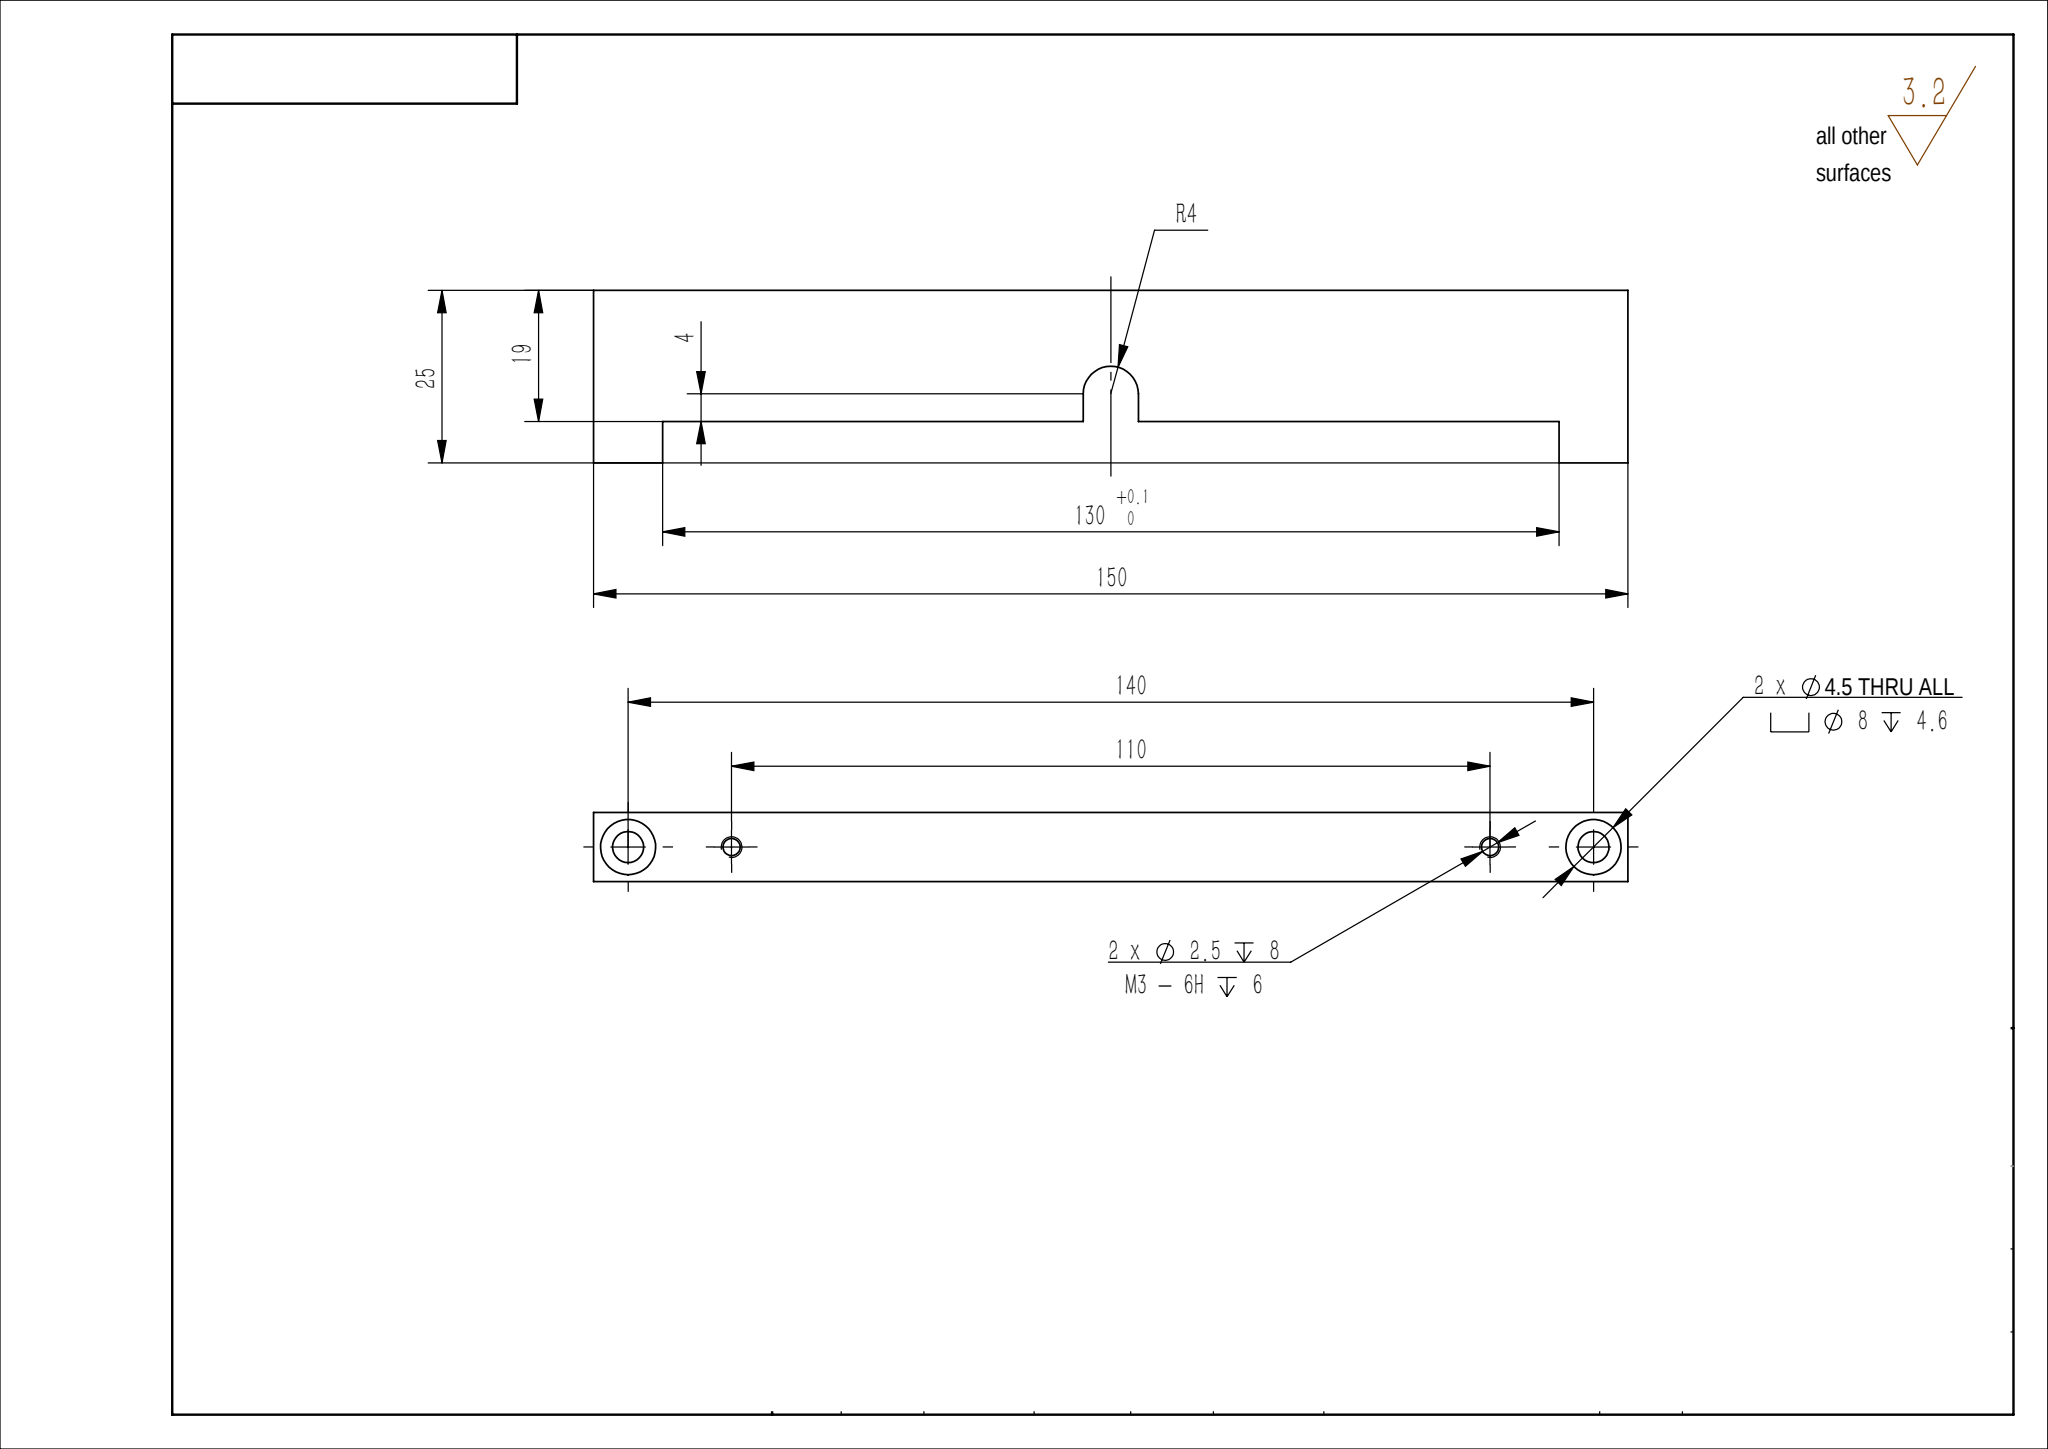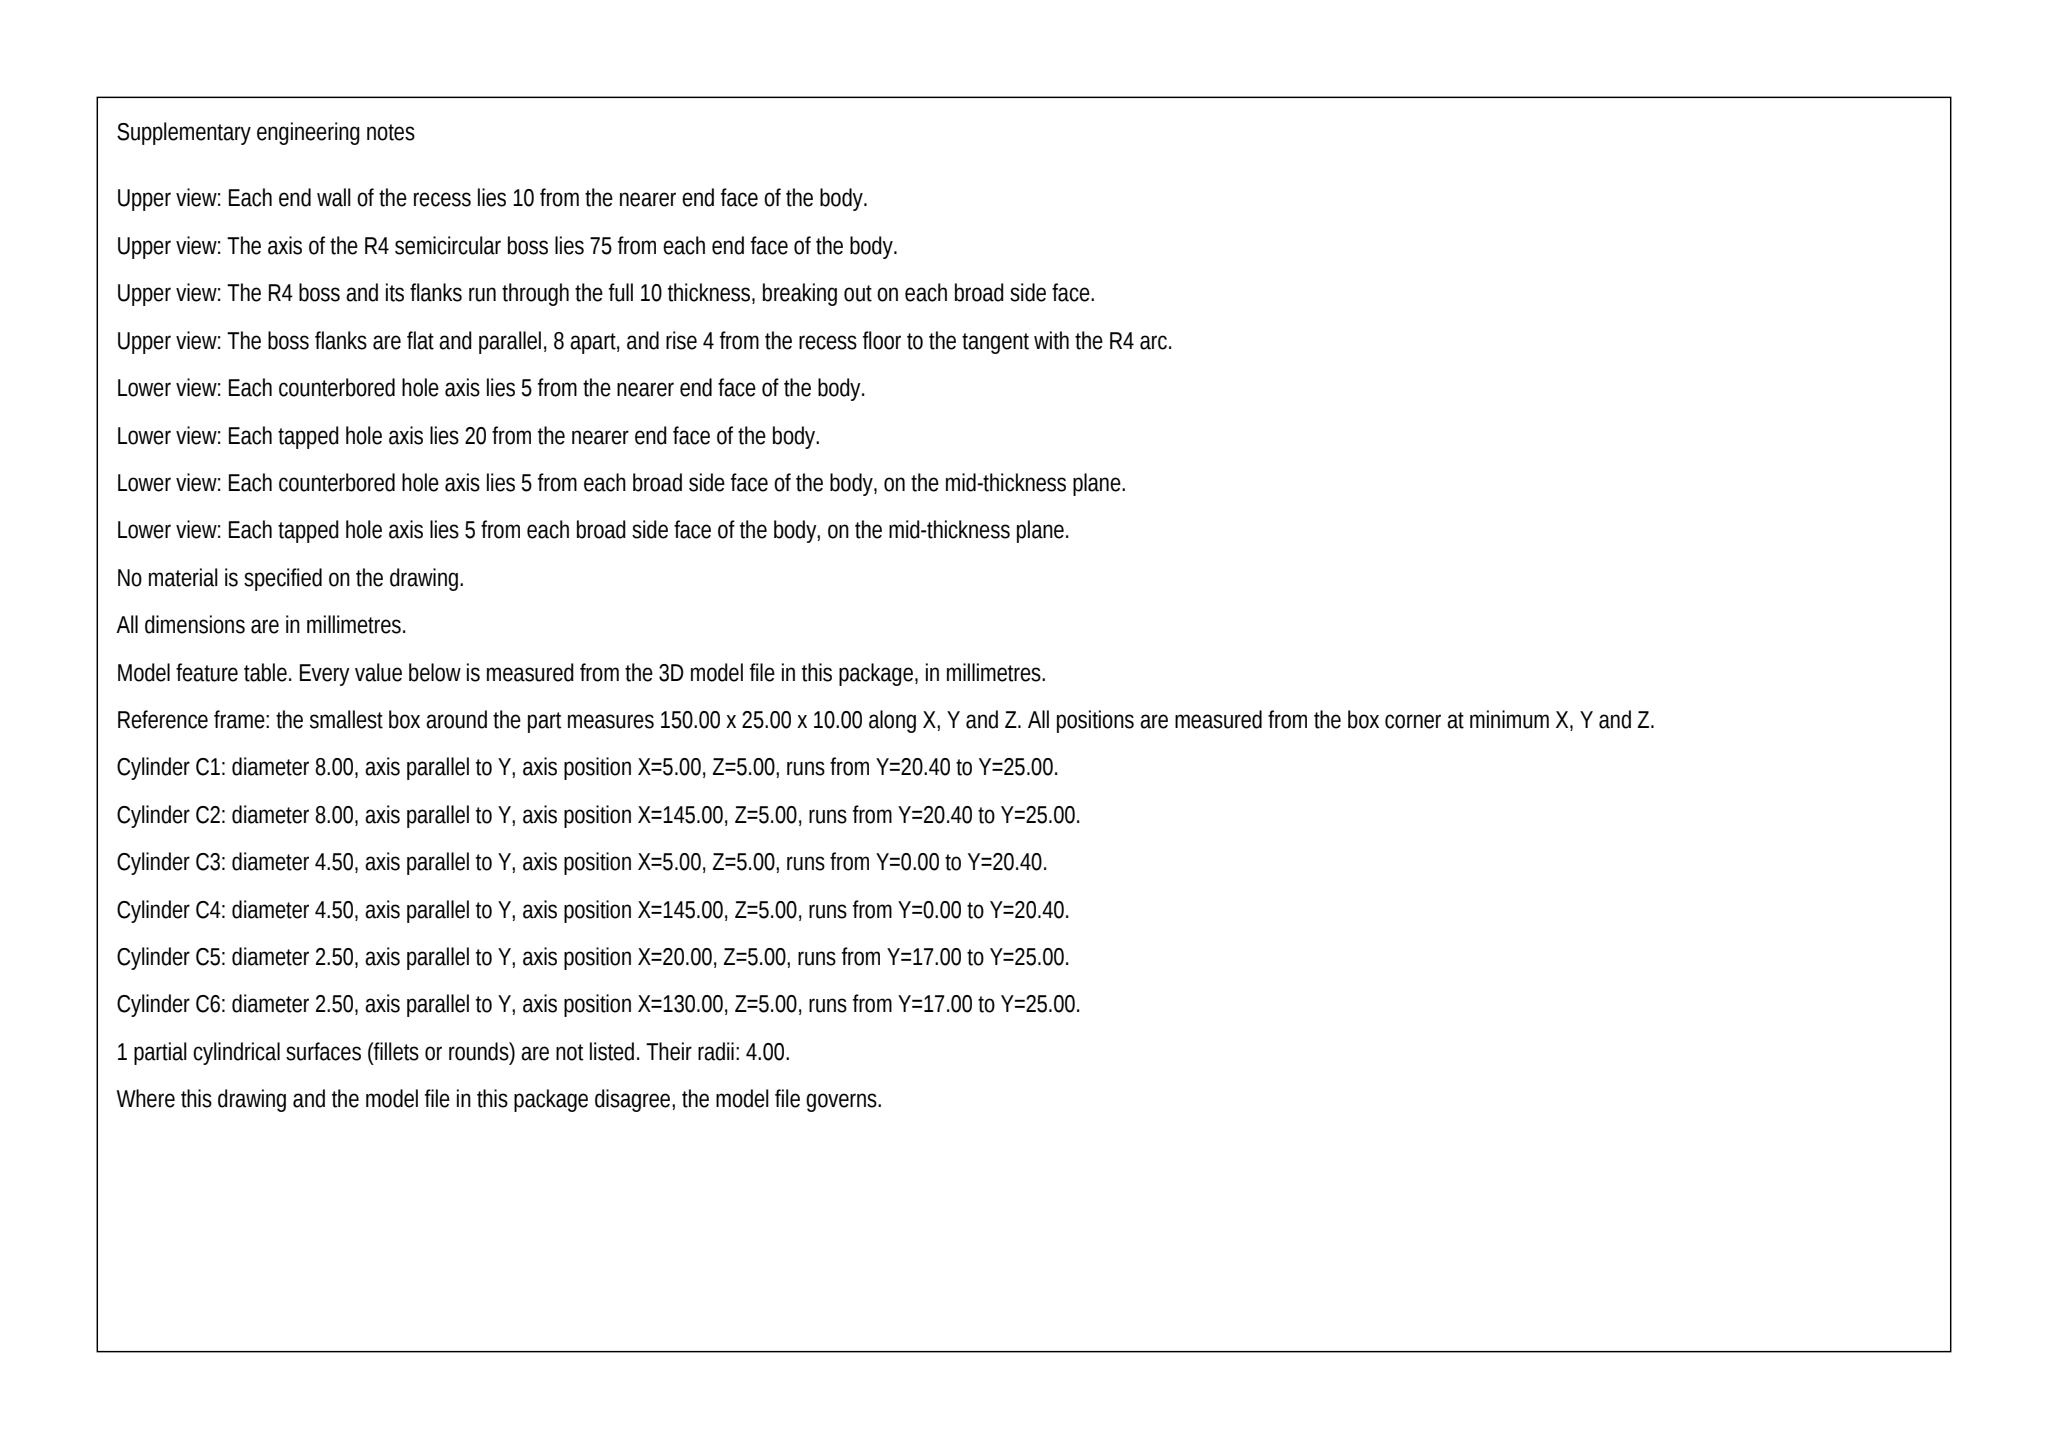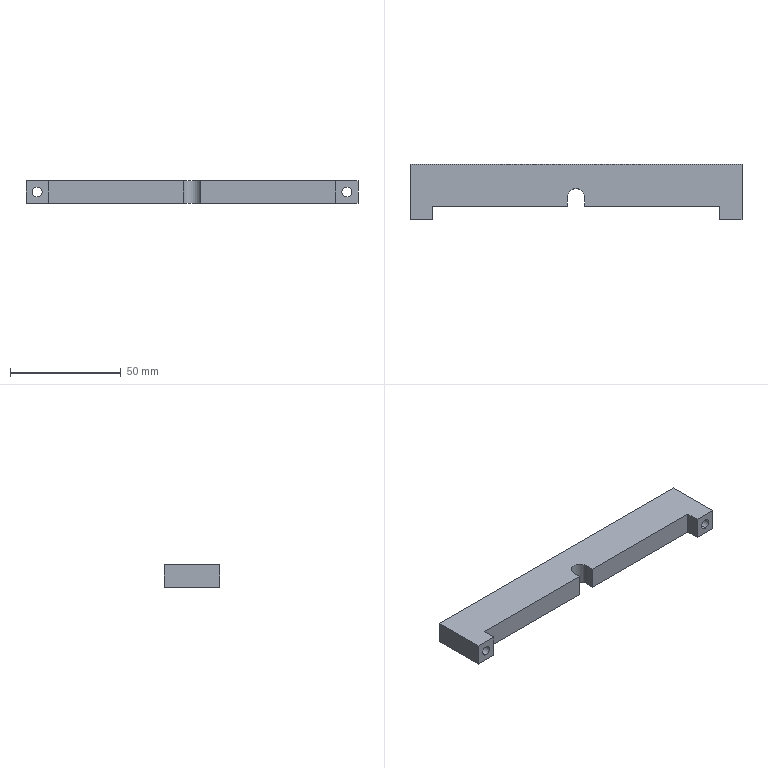Part | SolidWorks | mm | 1 solid | 32 faces | box 150 x 25 x 10 mm | volume 27936 mm3 | plane 15 | cylinder 13 | cone 4 | commonest cylinder face diameters 8 x5 2.5 x4 4.5 x4
Drawing notes:
PLAN VIEW: OVERALL THK 10 | from the solid: bbox_xyz Z = 10.0; planes z=0.0 and z=10.0
ALL HOLES ON CL OF 10 THK: 5 FROM EACH FACE | from the solid: cylinders dia 2.5/4.5/8 axis y at z=5.0, thickness 10
R4 NOTCH C/L 75 FROM EACH END, SYM ABOUT L/2 | from the solid: Ø8 z-axis cyl at x=75 (flanks x=71/79), bbox length 150
130 STEP SYM ABOUT L/2, 10 FROM EACH END | from the solid: x planes at 10.0 and 140.0 within 150 overall
2X Ø4.5 C'BORED HOLES 5 FROM EACH END, ON C/L OF 10 WIDTH | from the solid: Ø4.5/Ø8 axes at x=5 & x=145, z=5 of 10 thk
2X M3 HOLES 20 FROM EACH END, ON C/L OF 10 WIDTH | from the solid: Ø2.5 axes at x=20 & x=130, z=5 of 10 thk
Ø8 DP 4.6 C'BORE & M3 DP 6 FROM TOP FACE, OPP 130 STEP | from the solid: Ø8 c'bore y=20.4 to 25; step floor y=6, top face y=25
build123d program:
from build123d import *

# Parameters (mm, degrees)
SKETCH1_W                                         = 150
SKETCH1_H                                         = 10
BOSS_EXTRUDE1_DEPTH                               = 25
SKETCH2_W                                         = 130
SKETCH2_H                                         = 16.254
CUT_EXTRUDE1_DEPTH                                = 80.687
CUT_EXTRUDE2_DEPTH                                = 80.687
HOLE_SIZE_ACCORDING_TO_TYPE_1_HEXAGON_D           = 4.5
HOLE_SIZE_ACCORDING_TO_TYPE_1_HEXAGON_CBORE_D     = 8
HOLE_SIZE_ACCORDING_TO_TYPE_1_HEXAGON_CBORE_DEPTH = 4.6
M3_TAPPED_HOLE2_D                                 = 2.5
M3_TAPPED_HOLE2_DEPTH                             = 8
M3_TAPPED_HOLE2_TIP                               = 0.7511


with BuildPart() as part:
    # Sketch1 → Boss-Extrude1 (new body)
    with BuildSketch(Plane(origin=(0, 0, 0), x_dir=(1, 0, 0), z_dir=(0, 1, 0))):
        Rectangle(SKETCH1_W, SKETCH1_H)
    extrude(amount=BOSS_EXTRUDE1_DEPTH)

    # Sketch2 → Cut-Extrude1 (cut, through all)
    with BuildSketch(Plane.XY.offset(5)):
        with Locations((0, -2.127)):
            Rectangle(SKETCH2_W, SKETCH2_H)
    extrude(amount=-CUT_EXTRUDE1_DEPTH, mode=Mode.SUBTRACT)

    # Sketch3 → Cut-Extrude2 (cut, through all)
    with BuildSketch(Plane.XY.offset(5)):
        with BuildLine():
            Line((4, 10), (4, -5.136))
            ThreePointArc((4, -5.136), (0, -9.136), (-4, -5.136))
            Line((-4, -5.136), (-4, 10))
            ThreePointArc((-4, 10), (0, 14), (4, 10))
        make_face()
    extrude(amount=-CUT_EXTRUDE2_DEPTH, mode=Mode.SUBTRACT)

    # Hole Size _ according to_ Type 1 Hexagon (through all)
    with Locations(Plane(origin=(0, 25, 0), x_dir=(1, 0, 0), z_dir=(0, 1, 0))):
        with Locations((-70, 0), (70, 0)):
            CounterBoreHole(HOLE_SIZE_ACCORDING_TO_TYPE_1_HEXAGON_D / 2, HOLE_SIZE_ACCORDING_TO_TYPE_1_HEXAGON_CBORE_D / 2, HOLE_SIZE_ACCORDING_TO_TYPE_1_HEXAGON_CBORE_DEPTH)

    # M3 Tapped Hole2
    with Locations(Plane(origin=(0, 25, 0), x_dir=(1, 0, 0), z_dir=(0, 1, 0))):
        with Locations((55, 0), (-55, 0)):
            Hole(M3_TAPPED_HOLE2_D / 2, depth=M3_TAPPED_HOLE2_DEPTH)
            with Locations((0, 0, -(M3_TAPPED_HOLE2_DEPTH + M3_TAPPED_HOLE2_TIP / 2))):  # 118° drill point
                Cone(0, M3_TAPPED_HOLE2_D / 2, M3_TAPPED_HOLE2_TIP, mode=Mode.SUBTRACT)


solid = part.part